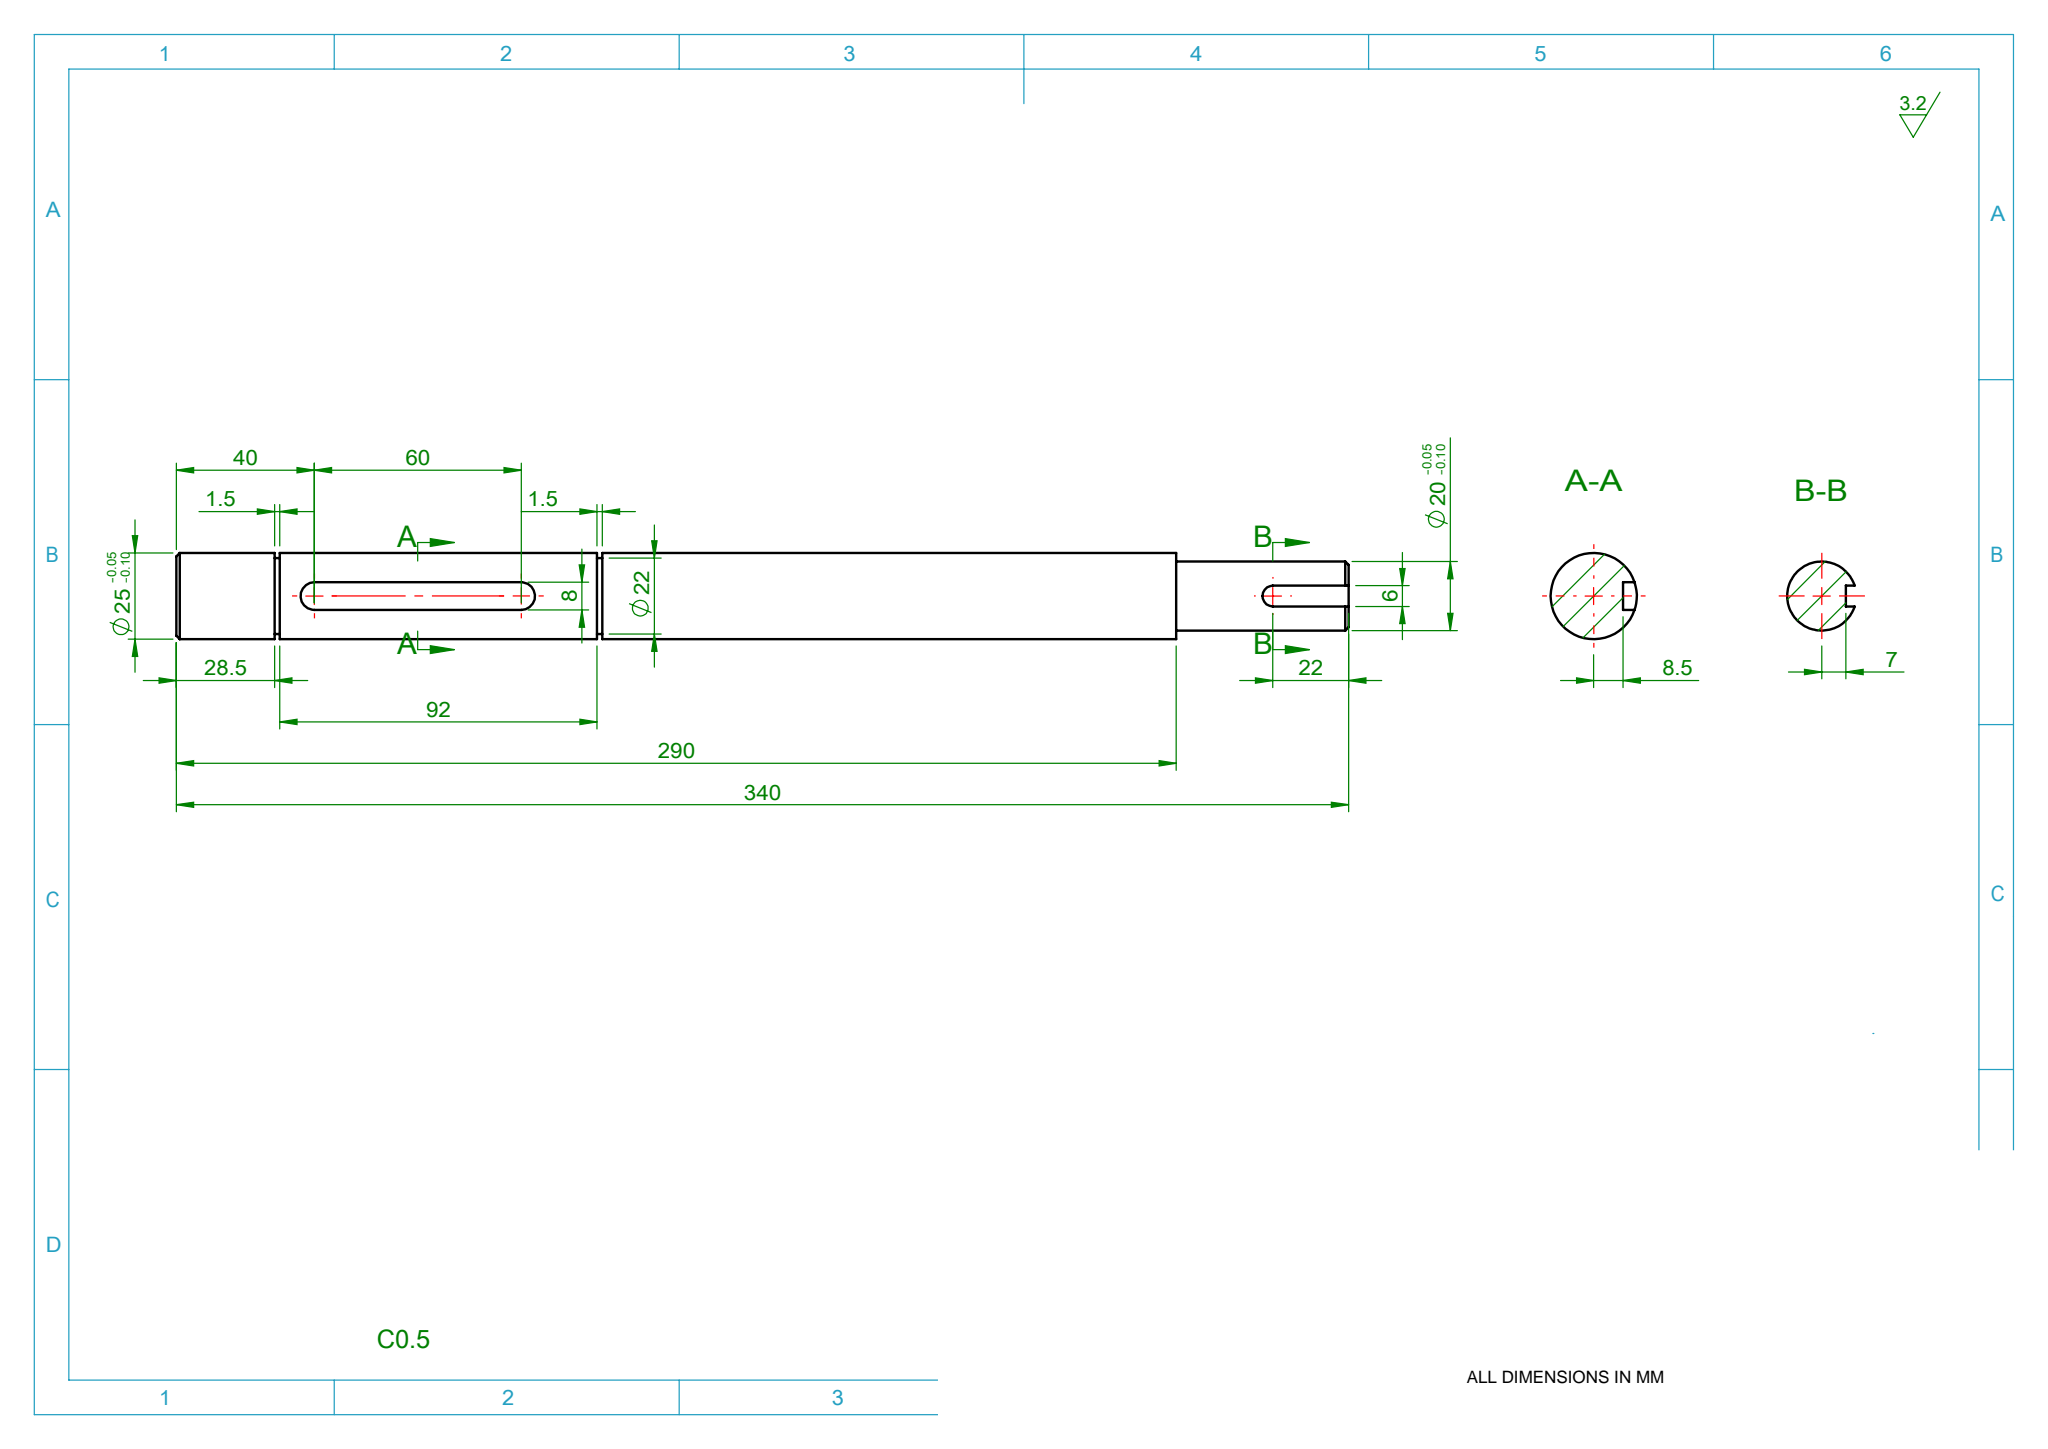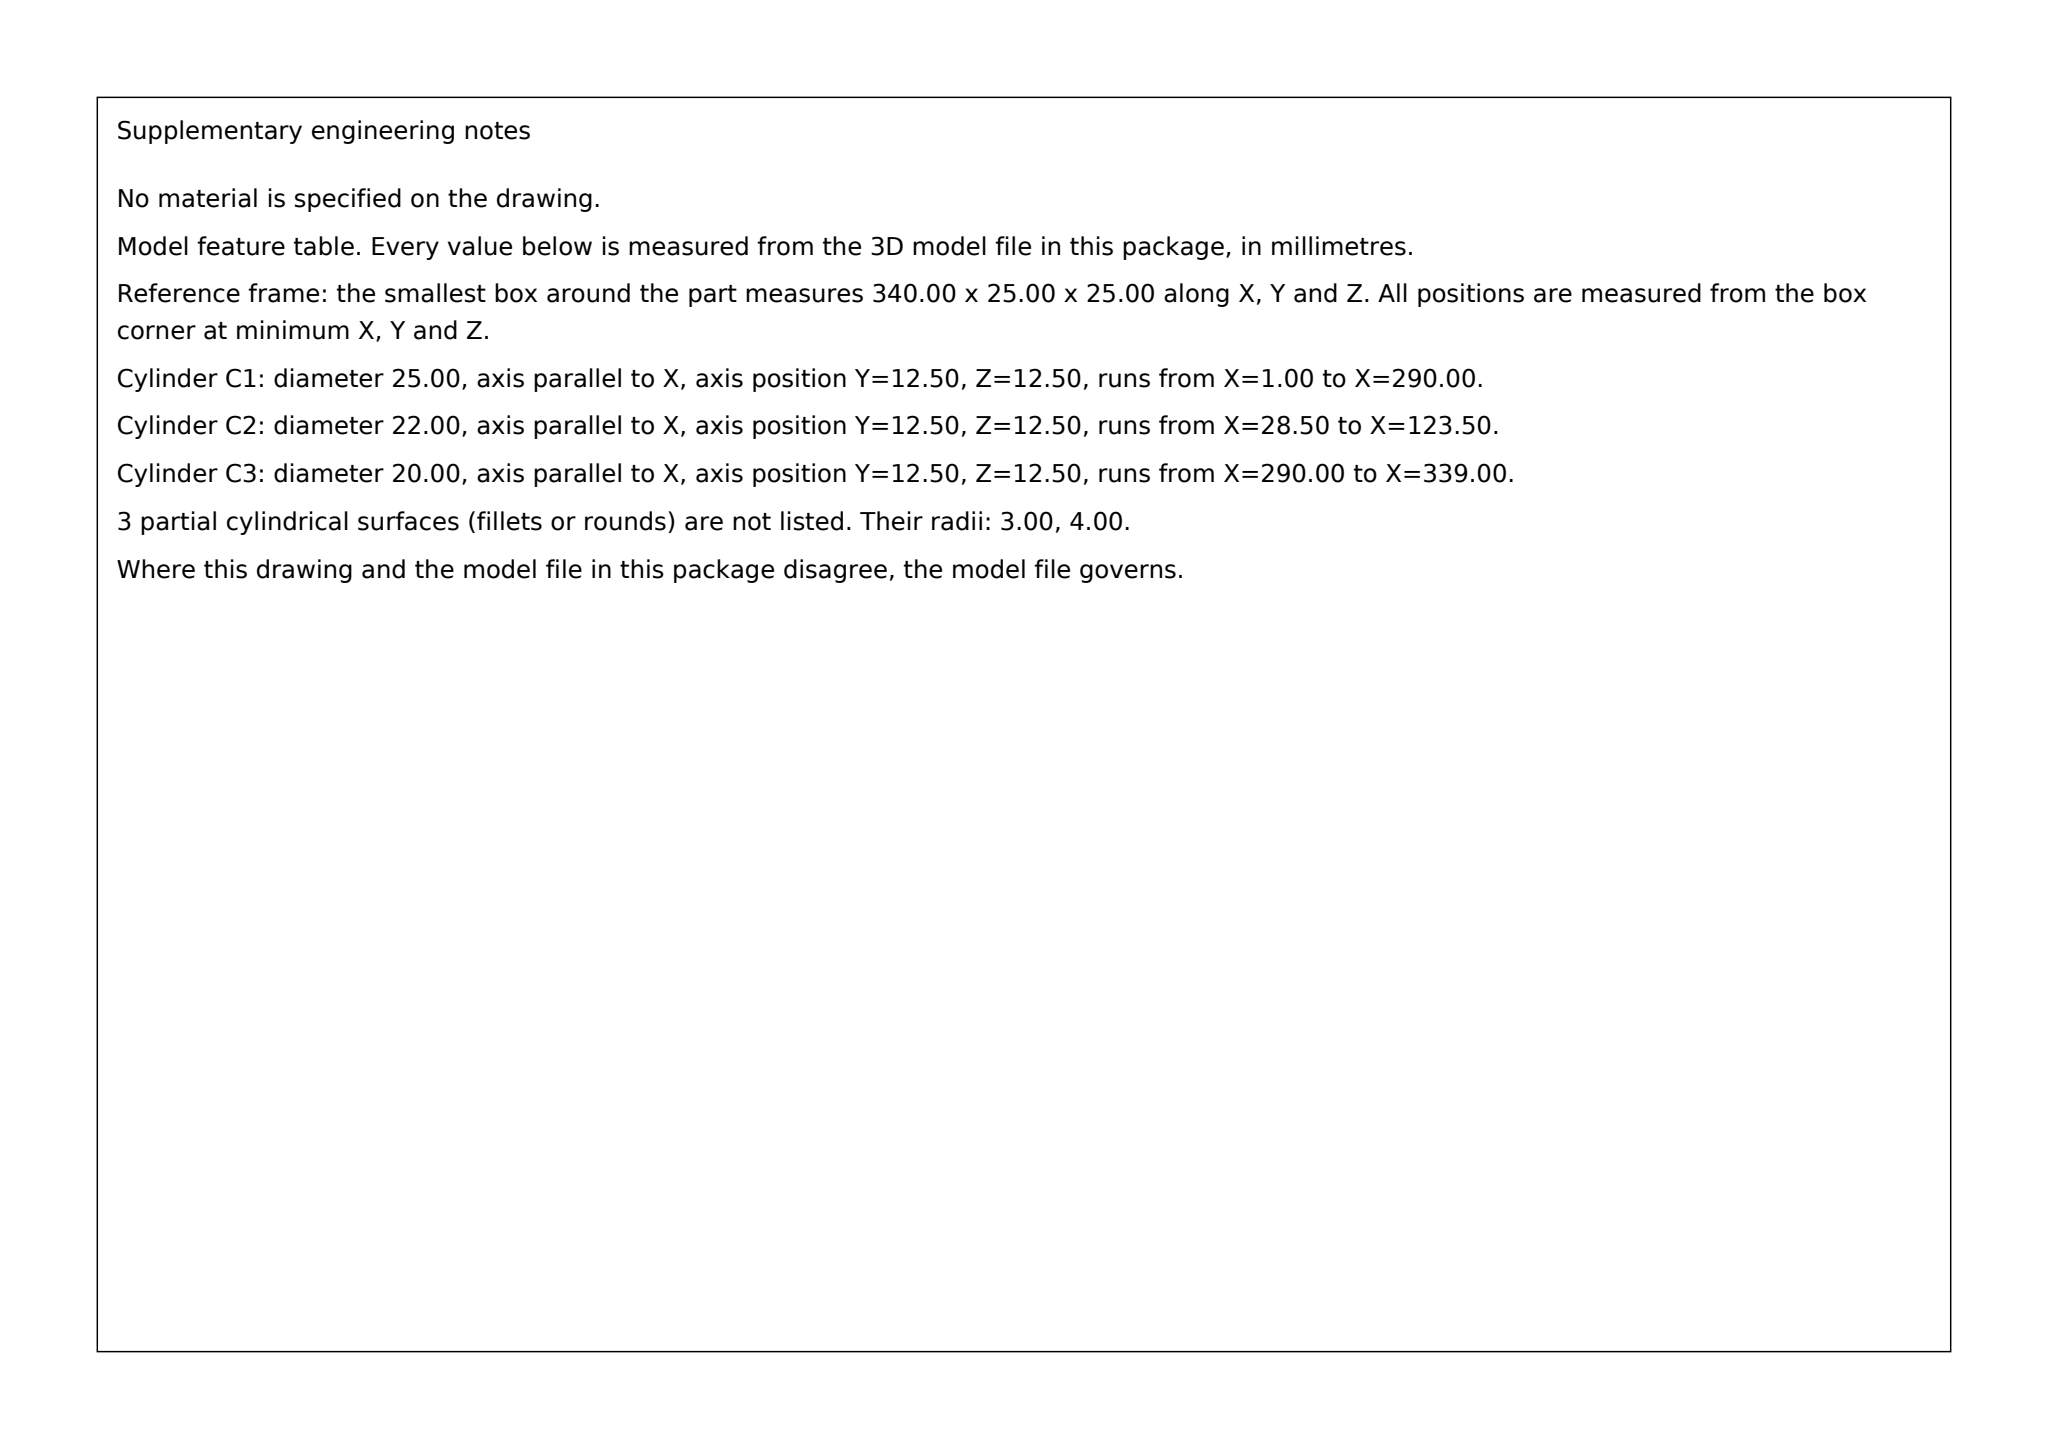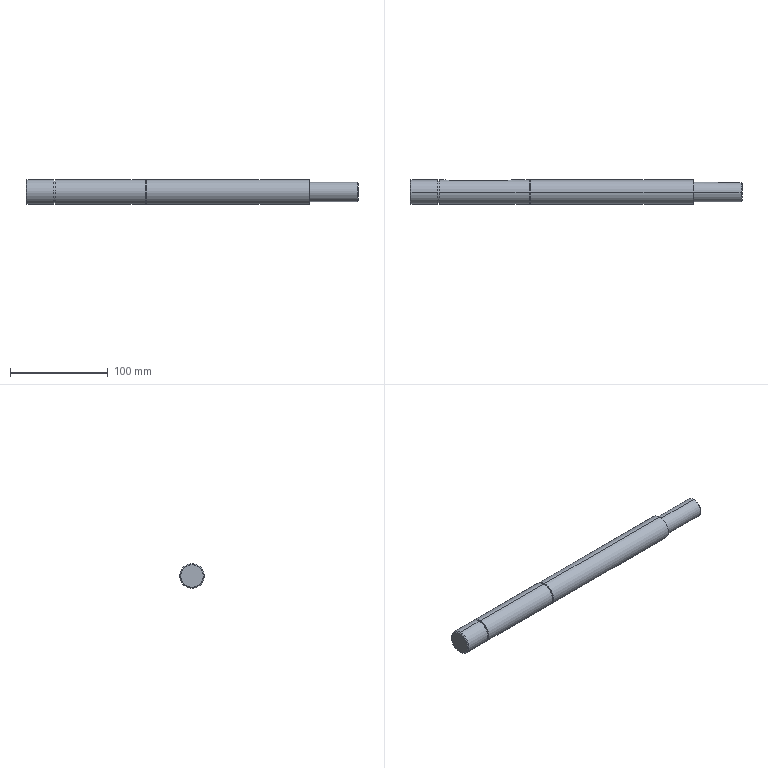Part | SolidWorks | mm | 1 solid | 34 faces | box 340 x 25 x 25 mm | volume 155238 mm3 | cylinder 16 | plane 13 | cone 5 | commonest cylinder face diameters 25 x6 22 x4 20 x2 8 x2 6 x2